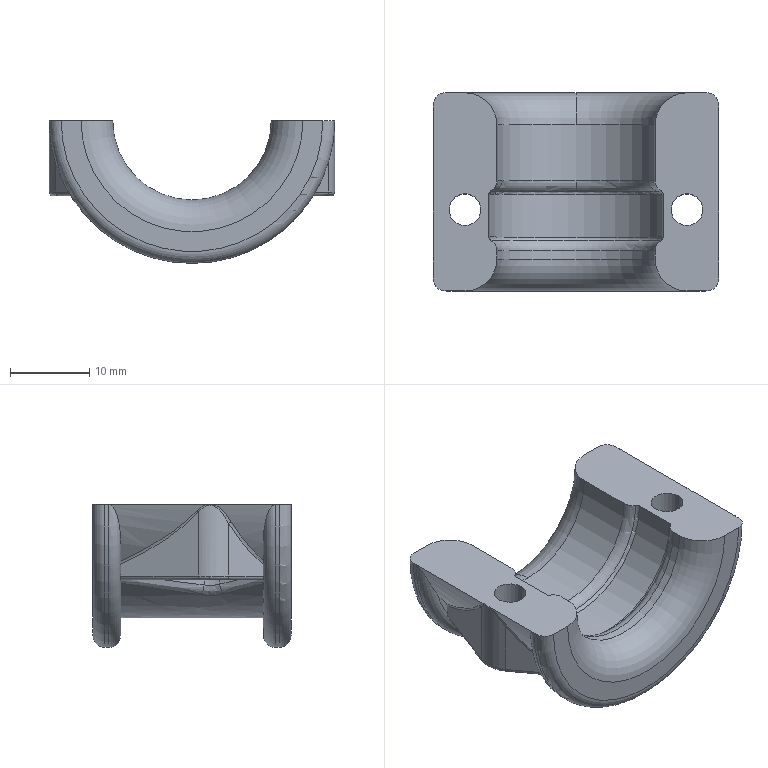Component | SolidWorks | Cache cable-1 | 1 solid | 84 faces | box 36 x 25 x 18 mm | volume 5929 mm3 | plane 24 | spline 24 | cylinder 19 | torus 17 | commonest cylinder face diameters 8 x6 4 x4 1 x4 20 x2 36 x2 22 x1